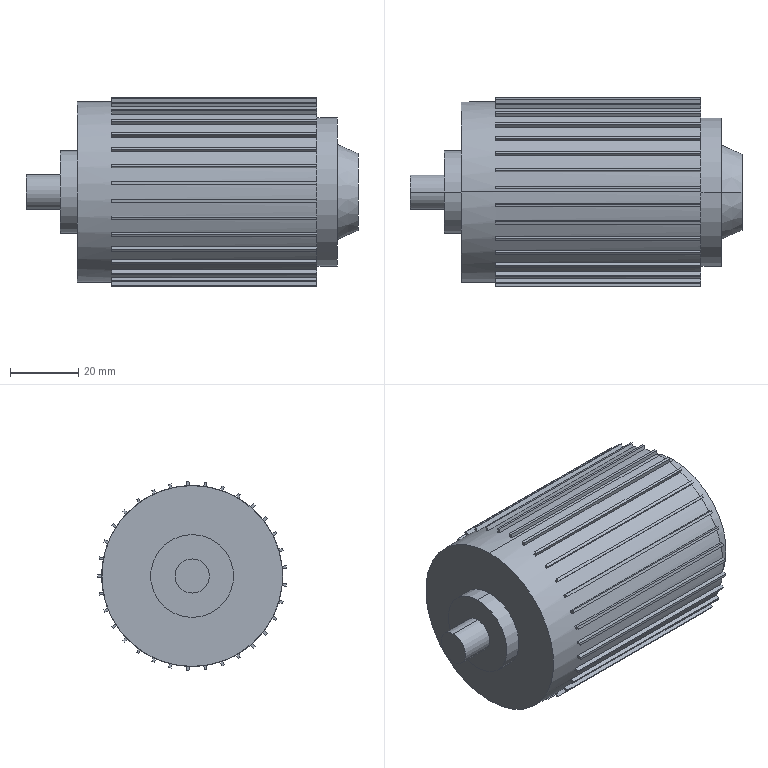Component | SolidWorks | Part10-1 | 1 solid | 148 faces | box 97 x 55.15 x 55.21 mm | volume 170335 mm3 | plane 138 | cylinder 8 | cone 2 | commonest cylinder face diameters 43.527 x2 52.845 x2 24.224 x2 10 x2
build123d program:
from build123d import *

# Parameters (mm, degrees)
SKETCH1_R           = 5
BOSS_EXTRUDE1_DEPTH = 10
SKETCH2_R           = 12.112
BOSS_EXTRUDE2_DEPTH = 5
SKETCH3_R           = 26.423
BOSS_EXTRUDE3_DEPTH = 70
SKETCH4_W           = 0.7635
SKETCH4_H           = 2.39
BOSS_EXTRUDE5_DEPTH = 60
CIRPATTERN1_COUNT   = 33
SKETCH5_R           = 21.764
BOSS_EXTRUDE6_DEPTH = 6
SKETCH6_R           = 13.88
BOSS_EXTRUDE7_DEPTH = 6
BOSS_EXTRUDE7_TAPER = 24


with BuildPart() as part:
    # Sketch1 → Boss-Extrude1 (new body)
    with BuildSketch(Plane.XY):
        with Locations((2289.28, 215.876)):
            Circle(SKETCH1_R)
    extrude(amount=BOSS_EXTRUDE1_DEPTH)

    # Sketch2 → Boss-Extrude2 (add)
    with BuildSketch(Plane.XY.offset(10)):
        with Locations((2289.28, 215.876)):
            Circle(SKETCH2_R)
    extrude(amount=BOSS_EXTRUDE2_DEPTH)

    # Sketch3 → Boss-Extrude3 (add)
    with BuildSketch(Plane.XY.offset(15)):
        with Locations((2289.28, 215.876)):
            Circle(SKETCH3_R)
    extrude(amount=BOSS_EXTRUDE3_DEPTH)

    # Sketch4 → Boss-Extrude5 (add)
    with BuildSketch(Plane.XY.offset(85)):
        with Locations((2289.28, 242.298)):
            Rectangle(SKETCH4_W, SKETCH4_H)
    boss_extrude5 = extrude(amount=-BOSS_EXTRUDE5_DEPTH)

    # CirPattern1: Boss-Extrude5 ×33 about axis
    cirpattern1_axis = Axis((2289.28, 215.876, 0), (0, 0, 1))
    for i in range(1, CIRPATTERN1_COUNT):
        add(boss_extrude5.rotate(cirpattern1_axis, i * 360 / CIRPATTERN1_COUNT))

    # Sketch5 → Boss-Extrude6 (add)
    with BuildSketch(Plane.XY.offset(85)):
        with Locations((2289.28, 215.876)):
            Circle(SKETCH5_R)
    extrude(amount=BOSS_EXTRUDE6_DEPTH)

    # Sketch6 → Boss-Extrude7 (add)
    with BuildSketch(Plane.XY.offset(91)):
        with Locations((2289.28, 215.876)):
            Circle(SKETCH6_R)
    extrude(amount=BOSS_EXTRUDE7_DEPTH, taper=BOSS_EXTRUDE7_TAPER)


solid = part.part

# Placed as in the assembly
solid = solid.moved(Location((152, 0, -143.093), (0, 90, 0)))